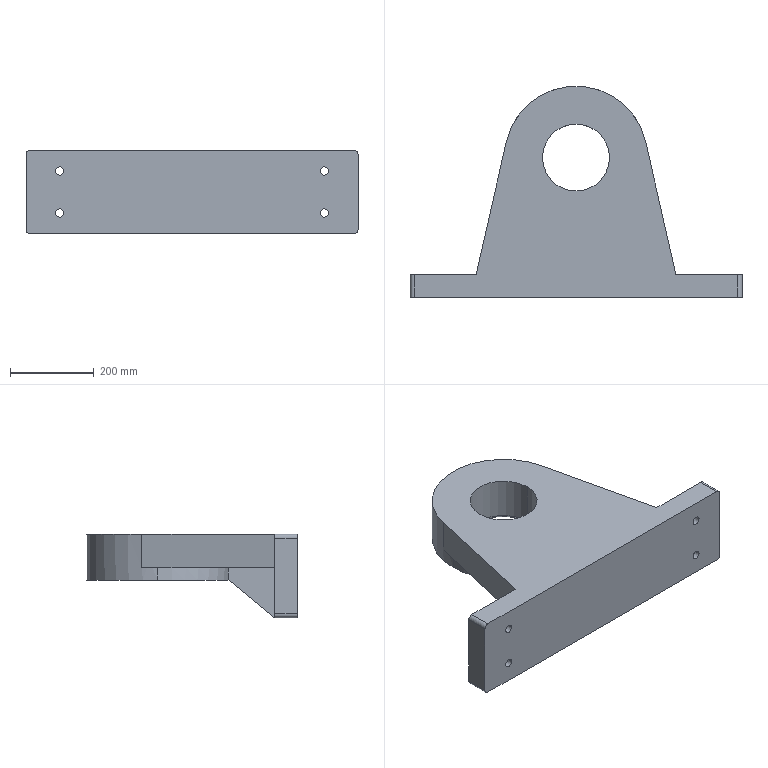Component | SolidWorks | SupportBase-1 | 1 solid | 34 faces | box 792.3 x 503.84 x 200 mm | volume 22321151 mm3 | cylinder 17 | plane 15 | cone 2 | commonest cylinder face diameters 20 x12 340.971 x3 160 x2 | material 45
STEP:
#1=CARTESIAN_POINT('',(57.666,-2.087,-8.071));
#2=VERTEX_POINT('',#1);
#3=CARTESIAN_POINT('',(56.878,-2.087,-8.071));
#4=VERTEX_POINT('',#3);
#5=CARTESIAN_POINT('',(57.272,-2.087,-8.071));
#6=DIRECTION('',(-0.,1.,0.));
#7=DIRECTION('',(-1.,0.,0.));
#8=AXIS2_PLACEMENT_3D('',#5,#6,#7);
#9=CIRCLE('',#8,0.3937);
#10=EDGE_CURVE('',#2,#4,#9,.T.);
#11=ORIENTED_EDGE('',*,*,#10,.F.);
#12=CARTESIAN_POINT('',(57.666,0.04869,-8.071));
#13=VERTEX_POINT('',#12);
#14=CARTESIAN_POINT('',(57.666,-5.424,-8.071));
#15=DIRECTION('',(-0.,1.,0.));
#16=VECTOR('',#15,39.37);
#17=LINE('',#14,#16);
#18=EDGE_CURVE('',#2,#13,#17,.T.);
#19=ORIENTED_EDGE('',*,*,#18,.T.);
#20=CARTESIAN_POINT('',(56.878,0.04869,-8.071));
#21=VERTEX_POINT('',#20);
#22=CARTESIAN_POINT('',(57.272,0.04869,-8.071));
#23=DIRECTION('',(-0.,1.,0.));
#24=DIRECTION('',(-1.,-0.,0.));
#25=AXIS2_PLACEMENT_3D('',#22,#23,#24);
#26=CIRCLE('',#25,0.3937);
#27=EDGE_CURVE('',#13,#21,#26,.T.);
#28=ORIENTED_EDGE('',*,*,#27,.T.);
#29=CARTESIAN_POINT('',(56.878,-5.424,-8.071));
#30=DIRECTION('',(-0.,1.,0.));
#31=VECTOR('',#30,39.37);
#32=LINE('',#29,#31);
#33=EDGE_CURVE('',#4,#21,#32,.T.);
#34=ORIENTED_EDGE('',*,*,#33,.F.);
#35=EDGE_LOOP('',(#11,#19,#28,#34));
#36=FACE_OUTER_BOUND('',#35,.T.);
#37=CARTESIAN_POINT('',(57.272,-5.424,-8.071));
#38=DIRECTION('',(-0.,1.,0.));
#39=DIRECTION('',(-1.,0.,0.));
#40=AXIS2_PLACEMENT_3D('',#37,#38,#39);
#41=CYLINDRICAL_SURFACE('',#40,0.3937);
#42=ADVANCED_FACE('',(#36),#41,.F.);
#43=CARTESIAN_POINT('',(57.666,-2.087,-12.008));
#44=VERTEX_POINT('',#43);
#45=CARTESIAN_POINT('',(56.878,-2.087,-12.008));
#46=VERTEX_POINT('',#45);
#47=CARTESIAN_POINT('',(57.272,-2.087,-12.008));
#48=DIRECTION('',(-0.,1.,0.));
#49=DIRECTION('',(-1.,0.,0.));
#50=AXIS2_PLACEMENT_3D('',#47,#48,#49);
#51=CIRCLE('',#50,0.3937);
#52=EDGE_CURVE('',#44,#46,#51,.T.);
#53=ORIENTED_EDGE('',*,*,#52,.F.);
#54=CARTESIAN_POINT('',(57.666,0.04869,-12.008));
#55=VERTEX_POINT('',#54);
#56=CARTESIAN_POINT('',(57.666,-5.424,-12.008));
#57=DIRECTION('',(-0.,1.,0.));
#58=VECTOR('',#57,39.37);
#59=LINE('',#56,#58);
#60=EDGE_CURVE('',#44,#55,#59,.T.);
#61=ORIENTED_EDGE('',*,*,#60,.T.);
#62=CARTESIAN_POINT('',(56.878,0.04869,-12.008));
#63=VERTEX_POINT('',#62);
#64=CARTESIAN_POINT('',(57.272,0.04869,-12.008));
#65=DIRECTION('',(-0.,1.,0.));
#66=DIRECTION('',(1.,0.,0.));
#67=AXIS2_PLACEMENT_3D('',#64,#65,#66);
#68=CIRCLE('',#67,0.3937);
#69=EDGE_CURVE('',#55,#63,#68,.T.);
#70=ORIENTED_EDGE('',*,*,#69,.T.);
#71=CARTESIAN_POINT('',(56.878,-5.424,-12.008));
#72=DIRECTION('',(-0.,1.,0.));
#73=VECTOR('',#72,39.37);
#74=LINE('',#71,#73);
#75=EDGE_CURVE('',#46,#63,#74,.T.);
#76=ORIENTED_EDGE('',*,*,#75,.F.);
#77=EDGE_LOOP('',(#53,#61,#70,#76));
#78=FACE_OUTER_BOUND('',#77,.T.);
#79=CARTESIAN_POINT('',(57.272,-5.424,-12.008));
#80=DIRECTION('',(-0.,1.,0.));
#81=DIRECTION('',(-1.,0.,0.));
#82=AXIS2_PLACEMENT_3D('',#79,#80,#81);
#83=CYLINDRICAL_SURFACE('',#82,0.3937);
#84=ADVANCED_FACE('',(#78),#83,.F.);
#85=CARTESIAN_POINT('',(32.772,-2.087,-8.071));
#86=VERTEX_POINT('',#85);
#87=CARTESIAN_POINT('',(31.985,-2.087,-8.071));
#88=VERTEX_POINT('',#87);
#89=CARTESIAN_POINT('',(32.378,-2.087,-8.071));
#90=DIRECTION('',(-0.,1.,0.));
#91=DIRECTION('',(-1.,0.,0.));
#92=AXIS2_PLACEMENT_3D('',#89,#90,#91);
#93=CIRCLE('',#92,0.3937);
#94=EDGE_CURVE('',#86,#88,#93,.T.);
#95=ORIENTED_EDGE('',*,*,#94,.F.);
#96=CARTESIAN_POINT('',(32.772,0.04869,-8.071));
#97=VERTEX_POINT('',#96);
#98=CARTESIAN_POINT('',(32.772,-5.424,-8.071));
#99=DIRECTION('',(-0.,1.,0.));
#100=VECTOR('',#99,39.37);
#101=LINE('',#98,#100);
#102=EDGE_CURVE('',#86,#97,#101,.T.);
#103=ORIENTED_EDGE('',*,*,#102,.T.);
#104=CARTESIAN_POINT('',(31.985,0.04869,-8.071));
#105=VERTEX_POINT('',#104);
#106=CARTESIAN_POINT('',(32.378,0.04869,-8.071));
#107=DIRECTION('',(-0.,1.,0.));
#108=DIRECTION('',(1.,0.,0.));
#109=AXIS2_PLACEMENT_3D('',#106,#107,#108);
#110=CIRCLE('',#109,0.3937);
#111=EDGE_CURVE('',#97,#105,#110,.T.);
#112=ORIENTED_EDGE('',*,*,#111,.T.);
#113=CARTESIAN_POINT('',(31.985,-5.424,-8.071));
#114=DIRECTION('',(-0.,1.,0.));
#115=VECTOR('',#114,39.37);
#116=LINE('',#113,#115);
#117=EDGE_CURVE('',#88,#105,#116,.T.);
#118=ORIENTED_EDGE('',*,*,#117,.F.);
#119=EDGE_LOOP('',(#95,#103,#112,#118));
#120=FACE_OUTER_BOUND('',#119,.T.);
#121=CARTESIAN_POINT('',(32.378,-5.424,-8.071));
#122=DIRECTION('',(-0.,1.,0.));
#123=DIRECTION('',(-1.,0.,0.));
#124=AXIS2_PLACEMENT_3D('',#121,#122,#123);
#125=CYLINDRICAL_SURFACE('',#124,0.3937);
#126=ADVANCED_FACE('',(#120),#125,.F.);
#127=CARTESIAN_POINT('',(32.772,-2.087,-12.008));
#128=VERTEX_POINT('',#127);
#129=CARTESIAN_POINT('',(31.985,-2.087,-12.008));
#130=VERTEX_POINT('',#129);
#131=CARTESIAN_POINT('',(32.378,-2.087,-12.008));
#132=DIRECTION('',(-0.,1.,0.));
#133=DIRECTION('',(-1.,0.,0.));
#134=AXIS2_PLACEMENT_3D('',#131,#132,#133);
#135=CIRCLE('',#134,0.3937);
#136=EDGE_CURVE('',#128,#130,#135,.T.);
#137=ORIENTED_EDGE('',*,*,#136,.F.);
#138=CARTESIAN_POINT('',(32.772,0.04869,-12.008));
#139=VERTEX_POINT('',#138);
#140=CARTESIAN_POINT('',(32.772,-5.424,-12.008));
#141=DIRECTION('',(-0.,1.,0.));
#142=VECTOR('',#141,39.37);
#143=LINE('',#140,#142);
#144=EDGE_CURVE('',#128,#139,#143,.T.);
#145=ORIENTED_EDGE('',*,*,#144,.T.);
#146=CARTESIAN_POINT('',(31.985,0.04869,-12.008));
#147=VERTEX_POINT('',#146);
#148=CARTESIAN_POINT('',(32.378,0.04869,-12.008));
#149=DIRECTION('',(-0.,1.,0.));
#150=DIRECTION('',(-1.,-0.,0.));
#151=AXIS2_PLACEMENT_3D('',#148,#149,#150);
#152=CIRCLE('',#151,0.3937);
#153=EDGE_CURVE('',#139,#147,#152,.T.);
#154=ORIENTED_EDGE('',*,*,#153,.T.);
#155=CARTESIAN_POINT('',(31.985,-5.424,-12.008));
#156=DIRECTION('',(-0.,1.,0.));
#157=VECTOR('',#156,39.37);
#158=LINE('',#155,#157);
#159=EDGE_CURVE('',#130,#147,#158,.T.);
#160=ORIENTED_EDGE('',*,*,#159,.F.);
#161=EDGE_LOOP('',(#137,#145,#154,#160));
#162=FACE_OUTER_BOUND('',#161,.T.);
#163=CARTESIAN_POINT('',(32.378,-5.424,-12.008));
#164=DIRECTION('',(-0.,1.,0.));
#165=DIRECTION('',(-1.,0.,0.));
#166=AXIS2_PLACEMENT_3D('',#163,#164,#165);
#167=CYLINDRICAL_SURFACE('',#166,0.3937);
#168=ADVANCED_FACE('',(#162),#167,.F.);
#169=CARTESIAN_POINT('',(47.975,11.038,-10.039));
#170=VERTEX_POINT('',#169);
#171=CARTESIAN_POINT('',(41.676,11.038,-10.039));
#172=VERTEX_POINT('',#171);
#173=CARTESIAN_POINT('',(44.825,11.038,-10.039));
#174=DIRECTION('',(0.,0.,-1.));
#175=DIRECTION('',(-1.,0.,0.));
#176=AXIS2_PLACEMENT_3D('',#173,#174,#175);
#177=CIRCLE('',#176,3.15);
#178=EDGE_CURVE('',#170,#172,#177,.T.);
#179=ORIENTED_EDGE('',*,*,#178,.F.);
#180=CARTESIAN_POINT('',(48.369,11.038,-10.433));
#181=VERTEX_POINT('',#180);
#182=CARTESIAN_POINT('',(47.975,11.038,-10.039));
#183=DIRECTION('',(0.7071,0.,-0.7071));
#184=VECTOR('',#183,39.37);
#185=LINE('',#182,#184);
#186=EDGE_CURVE('',#170,#181,#185,.T.);
#187=ORIENTED_EDGE('',*,*,#186,.T.);
#188=CARTESIAN_POINT('',(41.282,11.038,-10.433));
#189=VERTEX_POINT('',#188);
#190=CARTESIAN_POINT('',(44.825,11.038,-10.433));
#191=DIRECTION('',(0.,0.,1.));
#192=DIRECTION('',(-1.,0.,0.));
#193=AXIS2_PLACEMENT_3D('',#190,#191,#192);
#194=CIRCLE('',#193,3.543);
#195=EDGE_CURVE('',#189,#181,#194,.T.);
#196=ORIENTED_EDGE('',*,*,#195,.F.);
#197=CARTESIAN_POINT('',(41.676,11.038,-10.039));
#198=DIRECTION('',(-0.7071,0.,-0.7071));
#199=VECTOR('',#198,39.37);
#200=LINE('',#197,#199);
#201=EDGE_CURVE('',#172,#189,#200,.T.);
#202=ORIENTED_EDGE('',*,*,#201,.F.);
#203=EDGE_LOOP('',(#179,#187,#196,#202));
#204=FACE_OUTER_BOUND('',#203,.T.);
#205=CARTESIAN_POINT('',(44.825,11.038,-10.039));
#206=DIRECTION('',(0.,0.,-1.));
#207=DIRECTION('',(-1.,0.,0.));
#208=AXIS2_PLACEMENT_3D('',#205,#206,#207);
#209=CONICAL_SURFACE('',#208,3.15,0.7854);
#210=ADVANCED_FACE('',(#204),#209,.F.);
#211=CARTESIAN_POINT('',(41.676,11.038,-6.102));
#212=VERTEX_POINT('',#211);
#213=CARTESIAN_POINT('',(47.975,11.038,-6.102));
#214=VERTEX_POINT('',#213);
#215=CARTESIAN_POINT('',(44.825,11.038,-6.102));
#216=DIRECTION('',(0.,0.,1.));
#217=DIRECTION('',(1.,0.,0.));
#218=AXIS2_PLACEMENT_3D('',#215,#216,#217);
#219=CIRCLE('',#218,3.15);
#220=EDGE_CURVE('',#212,#214,#219,.T.);
#221=ORIENTED_EDGE('',*,*,#220,.T.);
#222=CARTESIAN_POINT('',(47.975,11.038,-6.102));
#223=DIRECTION('',(0.,0.,-1.));
#224=VECTOR('',#223,39.37);
#225=LINE('',#222,#224);
#226=EDGE_CURVE('',#214,#170,#225,.T.);
#227=ORIENTED_EDGE('',*,*,#226,.T.);
#228=ORIENTED_EDGE('',*,*,#178,.T.);
#229=CARTESIAN_POINT('',(41.676,11.038,-6.102));
#230=DIRECTION('',(0.,0.,-1.));
#231=VECTOR('',#230,39.37);
#232=LINE('',#229,#231);
#233=EDGE_CURVE('',#212,#172,#232,.T.);
#234=ORIENTED_EDGE('',*,*,#233,.F.);
#235=EDGE_LOOP('',(#221,#227,#228,#234));
#236=FACE_OUTER_BOUND('',#235,.T.);
#237=CARTESIAN_POINT('',(44.825,11.038,-6.102));
#238=DIRECTION('',(0.,0.,-1.));
#239=DIRECTION('',(-1.,0.,0.));
#240=AXIS2_PLACEMENT_3D('',#237,#238,#239);
#241=CYLINDRICAL_SURFACE('',#240,3.15);
#242=ADVANCED_FACE('',(#236),#241,.F.);
#243=CARTESIAN_POINT('',(51.37,12.528,-9.252));
#244=VERTEX_POINT('',#243);
#245=CARTESIAN_POINT('',(51.537,11.038,-9.252));
#246=VERTEX_POINT('',#245);
#247=CARTESIAN_POINT('',(44.825,11.038,-9.252));
#248=DIRECTION('',(0.,0.,-1.));
#249=DIRECTION('',(1.,0.,0.));
#250=AXIS2_PLACEMENT_3D('',#247,#248,#249);
#251=CIRCLE('',#250,6.712);
#252=EDGE_CURVE('',#244,#246,#251,.T.);
#253=ORIENTED_EDGE('',*,*,#252,.T.);
#254=CARTESIAN_POINT('',(51.537,11.038,-10.433));
#255=VERTEX_POINT('',#254);
#256=CARTESIAN_POINT('',(51.537,11.038,-6.102));
#257=DIRECTION('',(0.,0.,-1.));
#258=VECTOR('',#257,39.37);
#259=LINE('',#256,#258);
#260=EDGE_CURVE('',#246,#255,#259,.T.);
#261=ORIENTED_EDGE('',*,*,#260,.T.);
#262=CARTESIAN_POINT('',(38.113,11.038,-10.433));
#263=VERTEX_POINT('',#262);
#264=CARTESIAN_POINT('',(44.825,11.038,-10.433));
#265=DIRECTION('',(0.,0.,-1.));
#266=DIRECTION('',(-1.,0.,0.));
#267=AXIS2_PLACEMENT_3D('',#264,#265,#266);
#268=CIRCLE('',#267,6.712);
#269=EDGE_CURVE('',#263,#255,#268,.T.);
#270=ORIENTED_EDGE('',*,*,#269,.F.);
#271=CARTESIAN_POINT('',(38.113,11.038,-9.252));
#272=VERTEX_POINT('',#271);
#273=CARTESIAN_POINT('',(38.113,11.038,-6.102));
#274=DIRECTION('',(0.,0.,-1.));
#275=VECTOR('',#274,39.37);
#276=LINE('',#273,#275);
#277=EDGE_CURVE('',#272,#263,#276,.T.);
#278=ORIENTED_EDGE('',*,*,#277,.F.);
#279=CARTESIAN_POINT('',(38.281,12.528,-9.252));
#280=VERTEX_POINT('',#279);
#281=CARTESIAN_POINT('',(44.825,11.038,-9.252));
#282=DIRECTION('',(0.,0.,-1.));
#283=DIRECTION('',(1.,0.,0.));
#284=AXIS2_PLACEMENT_3D('',#281,#282,#283);
#285=CIRCLE('',#284,6.712);
#286=EDGE_CURVE('',#272,#280,#285,.T.);
#287=ORIENTED_EDGE('',*,*,#286,.T.);
#288=CARTESIAN_POINT('',(38.281,12.528,-6.102));
#289=VERTEX_POINT('',#288);
#290=CARTESIAN_POINT('',(38.281,12.528,-6.102));
#291=DIRECTION('',(0.,0.,-1.));
#292=VECTOR('',#291,39.37);
#293=LINE('',#290,#292);
#294=EDGE_CURVE('',#289,#280,#293,.T.);
#295=ORIENTED_EDGE('',*,*,#294,.F.);
#296=CARTESIAN_POINT('',(51.37,12.528,-6.102));
#297=VERTEX_POINT('',#296);
#298=CARTESIAN_POINT('',(44.825,11.038,-6.102));
#299=DIRECTION('',(0.,0.,1.));
#300=DIRECTION('',(1.,0.,0.));
#301=AXIS2_PLACEMENT_3D('',#298,#299,#300);
#302=CIRCLE('',#301,6.712);
#303=EDGE_CURVE('',#297,#289,#302,.T.);
#304=ORIENTED_EDGE('',*,*,#303,.F.);
#305=CARTESIAN_POINT('',(51.37,12.528,-6.102));
#306=DIRECTION('',(0.,0.,-1.));
#307=VECTOR('',#306,39.37);
#308=LINE('',#305,#307);
#309=EDGE_CURVE('',#297,#244,#308,.T.);
#310=ORIENTED_EDGE('',*,*,#309,.T.);
#311=EDGE_LOOP('',(#253,#261,#270,#278,#287,#295,#304,#310));
#312=FACE_OUTER_BOUND('',#311,.T.);
#313=CARTESIAN_POINT('',(44.825,11.038,-6.102));
#314=DIRECTION('',(0.,0.,-1.));
#315=DIRECTION('',(-1.,0.,0.));
#316=AXIS2_PLACEMENT_3D('',#313,#314,#315);
#317=CYLINDRICAL_SURFACE('',#316,6.712);
#318=ADVANCED_FACE('',(#312),#317,.T.);
#319=CARTESIAN_POINT('',(43.841,4.398,-9.252));
#320=VERTEX_POINT('',#319);
#321=CARTESIAN_POINT('',(44.825,11.038,-9.252));
#322=DIRECTION('',(0.,0.,-1.));
#323=DIRECTION('',(1.,0.,0.));
#324=AXIS2_PLACEMENT_3D('',#321,#322,#323);
#325=CIRCLE('',#324,6.712);
#326=EDGE_CURVE('',#320,#272,#325,.T.);
#327=ORIENTED_EDGE('',*,*,#326,.T.);
#328=ORIENTED_EDGE('',*,*,#277,.T.);
#329=CARTESIAN_POINT('',(44.825,4.326,-10.433));
#330=VERTEX_POINT('',#329);
#331=CARTESIAN_POINT('',(44.825,11.038,-10.433));
#332=DIRECTION('',(0.,0.,-1.));
#333=DIRECTION('',(-1.,0.,0.));
#334=AXIS2_PLACEMENT_3D('',#331,#332,#333);
#335=CIRCLE('',#334,6.712);
#336=EDGE_CURVE('',#330,#263,#335,.T.);
#337=ORIENTED_EDGE('',*,*,#336,.F.);
#338=CARTESIAN_POINT('',(43.841,4.398,-10.373));
#339=VERTEX_POINT('',#338);
#340=CARTESIAN_POINT('',(44.825,4.326,-10.433));
#341=CARTESIAN_POINT('',(44.496,4.326,-10.433));
#342=CARTESIAN_POINT('',(44.167,4.35,-10.413));
#343=CARTESIAN_POINT('',(43.841,4.398,-10.373));
#344=(BOUNDED_CURVE()B_SPLINE_CURVE(3,(#340,#341,#342,#343),.UNSPECIFIED.,.F.,.T.)B_SPLINE_CURVE_WITH_KNOTS((4,4),(0.,0.1472),.UNSPECIFIED.)CURVE()GEOMETRIC_REPRESENTATION_ITEM()RATIONAL_B_SPLINE_CURVE((1.,0.9982,0.9982,1.))REPRESENTATION_ITEM(''));
#345=EDGE_CURVE('',#330,#339,#344,.T.);
#346=ORIENTED_EDGE('',*,*,#345,.T.);
#347=CARTESIAN_POINT('',(43.841,4.398,-6.102));
#348=DIRECTION('',(0.,0.,1.));
#349=VECTOR('',#348,39.37);
#350=LINE('',#347,#349);
#351=EDGE_CURVE('',#339,#320,#350,.T.);
#352=ORIENTED_EDGE('',*,*,#351,.T.);
#353=EDGE_LOOP('',(#327,#328,#337,#346,#352));
#354=FACE_OUTER_BOUND('',#353,.T.);
#355=CARTESIAN_POINT('',(44.825,11.038,-6.102));
#356=DIRECTION('',(0.,0.,-1.));
#357=DIRECTION('',(-1.,0.,0.));
#358=AXIS2_PLACEMENT_3D('',#355,#356,#357);
#359=CYLINDRICAL_SURFACE('',#358,6.712);
#360=ADVANCED_FACE('',(#354),#359,.T.);
#361=CARTESIAN_POINT('',(45.81,4.398,-9.252));
#362=VERTEX_POINT('',#361);
#363=CARTESIAN_POINT('',(45.81,0.04869,-9.252));
#364=VERTEX_POINT('',#363);
#365=CARTESIAN_POINT('',(45.81,0.01034,-9.252));
#366=DIRECTION('',(0.,-1.,0.));
#367=VECTOR('',#366,39.37);
#368=LINE('',#365,#367);
#369=EDGE_CURVE('',#362,#364,#368,.T.);
#370=ORIENTED_EDGE('',*,*,#369,.F.);
#371=CARTESIAN_POINT('',(44.825,11.038,-9.252));
#372=DIRECTION('',(0.,0.,-1.));
#373=DIRECTION('',(1.,0.,0.));
#374=AXIS2_PLACEMENT_3D('',#371,#372,#373);
#375=CIRCLE('',#374,6.712);
#376=EDGE_CURVE('',#246,#362,#375,.T.);
#377=ORIENTED_EDGE('',*,*,#376,.F.);
#378=ORIENTED_EDGE('',*,*,#252,.F.);
#379=CARTESIAN_POINT('',(54.213,0.04869,-9.252));
#380=VERTEX_POINT('',#379);
#381=CARTESIAN_POINT('',(51.816,10.571,-9.252));
#382=DIRECTION('',(-0.2221,0.975,0.));
#383=VECTOR('',#382,39.37);
#384=LINE('',#381,#383);
#385=EDGE_CURVE('',#380,#244,#384,.T.);
#386=ORIENTED_EDGE('',*,*,#385,.F.);
#387=CARTESIAN_POINT('',(5.455,0.04869,-9.252));
#388=DIRECTION('',(-1.,0.,0.));
#389=VECTOR('',#388,39.37);
#390=LINE('',#387,#389);
#391=EDGE_CURVE('',#380,#364,#390,.T.);
#392=ORIENTED_EDGE('',*,*,#391,.T.);
#393=EDGE_LOOP('',(#370,#377,#378,#386,#392));
#394=FACE_OUTER_BOUND('',#393,.T.);
#395=CARTESIAN_POINT('',(5.455,0.01034,-9.252));
#396=DIRECTION('',(0.,0.,1.));
#397=DIRECTION('',(1.,0.,0.));
#398=AXIS2_PLACEMENT_3D('',#395,#396,#397);
#399=PLANE('',#398);
#400=ADVANCED_FACE('',(#394),#399,.F.);
#401=CARTESIAN_POINT('',(57.272,0.04869,-8.071));
#402=DIRECTION('',(-0.,1.,0.));
#403=DIRECTION('',(-1.,-0.,0.));
#404=AXIS2_PLACEMENT_3D('',#401,#402,#403);
#405=CIRCLE('',#404,0.3937);
#406=EDGE_CURVE('',#21,#13,#405,.T.);
#407=ORIENTED_EDGE('',*,*,#406,.F.);
#408=ORIENTED_EDGE('',*,*,#27,.F.);
#409=EDGE_LOOP('',(#407,#408));
#410=FACE_BOUND('',#409,.T.);
#411=CARTESIAN_POINT('',(57.272,0.04869,-12.008));
#412=DIRECTION('',(-0.,1.,0.));
#413=DIRECTION('',(1.,0.,0.));
#414=AXIS2_PLACEMENT_3D('',#411,#412,#413);
#415=CIRCLE('',#414,0.3937);
#416=EDGE_CURVE('',#63,#55,#415,.T.);
#417=ORIENTED_EDGE('',*,*,#416,.F.);
#418=ORIENTED_EDGE('',*,*,#69,.F.);
#419=EDGE_LOOP('',(#417,#418));
#420=FACE_BOUND('',#419,.T.);
#421=CARTESIAN_POINT('',(60.028,0.04869,-6.102));
#422=VERTEX_POINT('',#421);
#423=CARTESIAN_POINT('',(54.213,0.04869,-6.102));
#424=VERTEX_POINT('',#423);
#425=CARTESIAN_POINT('',(5.455,0.04869,-6.102));
#426=DIRECTION('',(-1.,-0.,0.));
#427=VECTOR('',#426,39.37);
#428=LINE('',#425,#427);
#429=EDGE_CURVE('',#422,#424,#428,.T.);
#430=ORIENTED_EDGE('',*,*,#429,.F.);
#431=CARTESIAN_POINT('',(60.422,0.04869,-6.496));
#432=VERTEX_POINT('',#431);
#433=CARTESIAN_POINT('',(60.028,0.04869,-6.496));
#434=DIRECTION('',(-0.,1.,0.));
#435=DIRECTION('',(1.,0.,0.));
#436=AXIS2_PLACEMENT_3D('',#433,#434,#435);
#437=CIRCLE('',#436,0.3937);
#438=EDGE_CURVE('',#422,#432,#437,.T.);
#439=ORIENTED_EDGE('',*,*,#438,.T.);
#440=CARTESIAN_POINT('',(60.422,0.04869,-13.583));
#441=VERTEX_POINT('',#440);
#442=CARTESIAN_POINT('',(60.422,0.04869,-6.102));
#443=DIRECTION('',(0.,0.,-1.));
#444=VECTOR('',#443,39.37);
#445=LINE('',#442,#444);
#446=EDGE_CURVE('',#432,#441,#445,.T.);
#447=ORIENTED_EDGE('',*,*,#446,.T.);
#448=CARTESIAN_POINT('',(60.028,0.04869,-13.976));
#449=VERTEX_POINT('',#448);
#450=CARTESIAN_POINT('',(60.028,0.04869,-13.583));
#451=DIRECTION('',(-0.,1.,0.));
#452=DIRECTION('',(1.,0.,0.));
#453=AXIS2_PLACEMENT_3D('',#450,#451,#452);
#454=CIRCLE('',#453,0.3937);
#455=EDGE_CURVE('',#441,#449,#454,.T.);
#456=ORIENTED_EDGE('',*,*,#455,.T.);
#457=CARTESIAN_POINT('',(45.81,0.04869,-13.976));
#458=VERTEX_POINT('',#457);
#459=CARTESIAN_POINT('',(29.229,0.04869,-13.976));
#460=DIRECTION('',(-1.,0.,0.));
#461=VECTOR('',#460,39.37);
#462=LINE('',#459,#461);
#463=EDGE_CURVE('',#449,#458,#462,.T.);
#464=ORIENTED_EDGE('',*,*,#463,.T.);
#465=CARTESIAN_POINT('',(45.81,0.04869,-6.102));
#466=DIRECTION('',(0.,0.,-1.));
#467=VECTOR('',#466,39.37);
#468=LINE('',#465,#467);
#469=EDGE_CURVE('',#364,#458,#468,.T.);
#470=ORIENTED_EDGE('',*,*,#469,.F.);
#471=ORIENTED_EDGE('',*,*,#391,.F.);
#472=CARTESIAN_POINT('',(54.213,0.04869,-6.102));
#473=DIRECTION('',(0.,0.,-1.));
#474=VECTOR('',#473,39.37);
#475=LINE('',#472,#474);
#476=EDGE_CURVE('',#424,#380,#475,.T.);
#477=ORIENTED_EDGE('',*,*,#476,.F.);
#478=EDGE_LOOP('',(#430,#439,#447,#456,#464,#470,#471,#477));
#479=FACE_OUTER_BOUND('',#478,.T.);
#480=CARTESIAN_POINT('',(5.455,0.04869,-6.102));
#481=DIRECTION('',(0.,-1.,0.));
#482=DIRECTION('',(1.,0.,0.));
#483=AXIS2_PLACEMENT_3D('',#480,#481,#482);
#484=PLANE('',#483);
#485=ADVANCED_FACE('',(#410,#420,#479),#484,.F.);
#486=ORIENTED_EDGE('',*,*,#326,.F.);
#487=CARTESIAN_POINT('',(43.841,0.04869,-9.252));
#488=VERTEX_POINT('',#487);
#489=CARTESIAN_POINT('',(43.841,0.01034,-9.252));
#490=DIRECTION('',(0.,-1.,0.));
#491=VECTOR('',#490,39.37);
#492=LINE('',#489,#491);
#493=EDGE_CURVE('',#320,#488,#492,.T.);
#494=ORIENTED_EDGE('',*,*,#493,.T.);
#495=CARTESIAN_POINT('',(35.438,0.04869,-9.252));
#496=VERTEX_POINT('',#495);
#497=CARTESIAN_POINT('',(5.455,0.04869,-9.252));
#498=DIRECTION('',(-1.,0.,0.));
#499=VECTOR('',#498,39.37);
#500=LINE('',#497,#499);
#501=EDGE_CURVE('',#488,#496,#500,.T.);
#502=ORIENTED_EDGE('',*,*,#501,.T.);
#503=CARTESIAN_POINT('',(33.951,-6.481,-9.252));
#504=DIRECTION('',(0.2221,0.975,0.));
#505=VECTOR('',#504,39.37);
#506=LINE('',#503,#505);
#507=EDGE_CURVE('',#496,#280,#506,.T.);
#508=ORIENTED_EDGE('',*,*,#507,.T.);
#509=ORIENTED_EDGE('',*,*,#286,.F.);
#510=EDGE_LOOP('',(#486,#494,#502,#508,#509));
#511=FACE_OUTER_BOUND('',#510,.T.);
#512=CARTESIAN_POINT('',(5.455,0.01034,-9.252));
#513=DIRECTION('',(0.,0.,1.));
#514=DIRECTION('',(1.,0.,0.));
#515=AXIS2_PLACEMENT_3D('',#512,#513,#514);
#516=PLANE('',#515);
#517=ADVANCED_FACE('',(#511),#516,.F.);
#518=ORIENTED_EDGE('',*,*,#260,.F.);
#519=ORIENTED_EDGE('',*,*,#376,.T.);
#520=CARTESIAN_POINT('',(45.81,4.398,-10.373));
#521=VERTEX_POINT('',#520);
#522=CARTESIAN_POINT('',(45.81,4.398,-6.102));
#523=DIRECTION('',(0.,0.,1.));
#524=VECTOR('',#523,39.37);
#525=LINE('',#522,#524);
#526=EDGE_CURVE('',#521,#362,#525,.T.);
#527=ORIENTED_EDGE('',*,*,#526,.F.);
#528=CARTESIAN_POINT('',(45.81,4.398,-10.373));
#529=CARTESIAN_POINT('',(45.484,4.35,-10.413));
#530=CARTESIAN_POINT('',(45.155,4.326,-10.433));
#531=CARTESIAN_POINT('',(44.825,4.326,-10.433));
#532=(BOUNDED_CURVE()B_SPLINE_CURVE(3,(#528,#529,#530,#531),.UNSPECIFIED.,.F.,.T.)B_SPLINE_CURVE_WITH_KNOTS((4,4),(6.136,6.283),.UNSPECIFIED.)CURVE()GEOMETRIC_REPRESENTATION_ITEM()RATIONAL_B_SPLINE_CURVE((1.,0.9982,0.9982,1.))REPRESENTATION_ITEM(''));
#533=EDGE_CURVE('',#521,#330,#532,.T.);
#534=ORIENTED_EDGE('',*,*,#533,.T.);
#535=CARTESIAN_POINT('',(44.825,11.038,-10.433));
#536=DIRECTION('',(0.,0.,-1.));
#537=DIRECTION('',(-1.,0.,0.));
#538=AXIS2_PLACEMENT_3D('',#535,#536,#537);
#539=CIRCLE('',#538,6.712);
#540=EDGE_CURVE('',#255,#330,#539,.T.);
#541=ORIENTED_EDGE('',*,*,#540,.F.);
#542=EDGE_LOOP('',(#518,#519,#527,#534,#541));
#543=FACE_OUTER_BOUND('',#542,.T.);
#544=CARTESIAN_POINT('',(44.825,11.038,-6.102));
#545=DIRECTION('',(0.,0.,-1.));
#546=DIRECTION('',(-1.,0.,0.));
#547=AXIS2_PLACEMENT_3D('',#544,#545,#546);
#548=CYLINDRICAL_SURFACE('',#547,6.712);
#549=ADVANCED_FACE('',(#543),#548,.T.);
#550=ORIENTED_EDGE('',*,*,#507,.F.);
#551=CARTESIAN_POINT('',(35.438,0.04869,-6.102));
#552=VERTEX_POINT('',#551);
#553=CARTESIAN_POINT('',(35.438,0.04869,-6.102));
#554=DIRECTION('',(0.,0.,-1.));
#555=VECTOR('',#554,39.37);
#556=LINE('',#553,#555);
#557=EDGE_CURVE('',#552,#496,#556,.T.);
#558=ORIENTED_EDGE('',*,*,#557,.F.);
#559=CARTESIAN_POINT('',(33.951,-6.481,-6.102));
#560=DIRECTION('',(0.2221,0.975,0.));
#561=VECTOR('',#560,39.37);
#562=LINE('',#559,#561);
#563=EDGE_CURVE('',#552,#289,#562,.T.);
#564=ORIENTED_EDGE('',*,*,#563,.T.);
#565=ORIENTED_EDGE('',*,*,#294,.T.);
#566=EDGE_LOOP('',(#550,#558,#564,#565));
#567=FACE_OUTER_BOUND('',#566,.T.);
#568=CARTESIAN_POINT('',(33.951,-6.481,-6.102));
#569=DIRECTION('',(-0.975,0.2221,0.));
#570=DIRECTION('',(-0.2221,-0.975,0.));
#571=AXIS2_PLACEMENT_3D('',#568,#569,#570);
#572=PLANE('',#571);
#573=ADVANCED_FACE('',(#567),#572,.T.);
#574=CARTESIAN_POINT('',(29.229,-2.087,-6.496));
#575=VERTEX_POINT('',#574);
#576=CARTESIAN_POINT('',(29.229,-2.087,-13.583));
#577=VERTEX_POINT('',#576);
#578=CARTESIAN_POINT('',(29.229,-2.087,-6.102));
#579=DIRECTION('',(0.,0.,-1.));
#580=VECTOR('',#579,39.37);
#581=LINE('',#578,#580);
#582=EDGE_CURVE('',#575,#577,#581,.T.);
#583=ORIENTED_EDGE('',*,*,#582,.F.);
#584=CARTESIAN_POINT('',(29.229,0.04869,-6.496));
#585=VERTEX_POINT('',#584);
#586=CARTESIAN_POINT('',(29.229,0.01034,-6.496));
#587=DIRECTION('',(0.,1.,0.));
#588=VECTOR('',#587,39.37);
#589=LINE('',#586,#588);
#590=EDGE_CURVE('',#575,#585,#589,.T.);
#591=ORIENTED_EDGE('',*,*,#590,.T.);
#592=CARTESIAN_POINT('',(29.229,0.04869,-13.583));
#593=VERTEX_POINT('',#592);
#594=CARTESIAN_POINT('',(29.229,0.04869,-6.102));
#595=DIRECTION('',(0.,0.,-1.));
#596=VECTOR('',#595,39.37);
#597=LINE('',#594,#596);
#598=EDGE_CURVE('',#585,#593,#597,.T.);
#599=ORIENTED_EDGE('',*,*,#598,.T.);
#600=CARTESIAN_POINT('',(29.229,-2.087,-13.583));
#601=DIRECTION('',(0.,-1.,0.));
#602=VECTOR('',#601,39.37);
#603=LINE('',#600,#602);
#604=EDGE_CURVE('',#593,#577,#603,.T.);
#605=ORIENTED_EDGE('',*,*,#604,.T.);
#606=EDGE_LOOP('',(#583,#591,#599,#605));
#607=FACE_OUTER_BOUND('',#606,.T.);
#608=CARTESIAN_POINT('',(29.229,0.01034,-6.102));
#609=DIRECTION('',(-1.,0.,0.));
#610=DIRECTION('',(0.,0.,1.));
#611=AXIS2_PLACEMENT_3D('',#608,#609,#610);
#612=PLANE('',#611);
#613=ADVANCED_FACE('',(#607),#612,.T.);
#614=CARTESIAN_POINT('',(32.378,-2.087,-8.071));
#615=DIRECTION('',(-0.,1.,0.));
#616=DIRECTION('',(-1.,0.,0.));
#617=AXIS2_PLACEMENT_3D('',#614,#615,#616);
#618=CIRCLE('',#617,0.3937);
#619=EDGE_CURVE('',#88,#86,#618,.T.);
#620=ORIENTED_EDGE('',*,*,#619,.T.);
#621=ORIENTED_EDGE('',*,*,#94,.T.);
#622=EDGE_LOOP('',(#620,#621));
#623=FACE_BOUND('',#622,.T.);
#624=CARTESIAN_POINT('',(57.272,-2.087,-8.071));
#625=DIRECTION('',(-0.,1.,0.));
#626=DIRECTION('',(-1.,0.,0.));
#627=AXIS2_PLACEMENT_3D('',#624,#625,#626);
#628=CIRCLE('',#627,0.3937);
#629=EDGE_CURVE('',#4,#2,#628,.T.);
#630=ORIENTED_EDGE('',*,*,#629,.T.);
#631=ORIENTED_EDGE('',*,*,#10,.T.);
#632=EDGE_LOOP('',(#630,#631));
#633=FACE_BOUND('',#632,.T.);
#634=CARTESIAN_POINT('',(57.272,-2.087,-12.008));
#635=DIRECTION('',(-0.,1.,0.));
#636=DIRECTION('',(-1.,0.,0.));
#637=AXIS2_PLACEMENT_3D('',#634,#635,#636);
#638=CIRCLE('',#637,0.3937);
#639=EDGE_CURVE('',#46,#44,#638,.T.);
#640=ORIENTED_EDGE('',*,*,#639,.T.);
#641=ORIENTED_EDGE('',*,*,#52,.T.);
#642=EDGE_LOOP('',(#640,#641));
#643=FACE_BOUND('',#642,.T.);
#644=CARTESIAN_POINT('',(32.378,-2.087,-12.008));
#645=DIRECTION('',(-0.,1.,0.));
#646=DIRECTION('',(-1.,0.,0.));
#647=AXIS2_PLACEMENT_3D('',#644,#645,#646);
#648=CIRCLE('',#647,0.3937);
#649=EDGE_CURVE('',#130,#128,#648,.T.);
#650=ORIENTED_EDGE('',*,*,#649,.T.);
#651=ORIENTED_EDGE('',*,*,#136,.T.);
#652=EDGE_LOOP('',(#650,#651));
#653=FACE_BOUND('',#652,.T.);
#654=CARTESIAN_POINT('',(60.422,-2.087,-6.496));
#655=VERTEX_POINT('',#654);
#656=CARTESIAN_POINT('',(60.422,-2.087,-13.583));
#657=VERTEX_POINT('',#656);
#658=CARTESIAN_POINT('',(60.422,-2.087,-6.102));
#659=DIRECTION('',(0.,0.,-1.));
#660=VECTOR('',#659,39.37);
#661=LINE('',#658,#660);
#662=EDGE_CURVE('',#655,#657,#661,.T.);
#663=ORIENTED_EDGE('',*,*,#662,.F.);
#664=CARTESIAN_POINT('',(60.028,-2.087,-6.102));
#665=VERTEX_POINT('',#664);
#666=CARTESIAN_POINT('',(60.028,-2.087,-6.496));
#667=DIRECTION('',(0.,-1.,0.));
#668=DIRECTION('',(-1.,0.,0.));
#669=AXIS2_PLACEMENT_3D('',#666,#667,#668);
#670=CIRCLE('',#669,0.3937);
#671=EDGE_CURVE('',#655,#665,#670,.T.);
#672=ORIENTED_EDGE('',*,*,#671,.T.);
#673=CARTESIAN_POINT('',(29.623,-2.087,-6.102));
#674=VERTEX_POINT('',#673);
#675=CARTESIAN_POINT('',(5.455,-2.087,-6.102));
#676=DIRECTION('',(1.,0.,0.));
#677=VECTOR('',#676,39.37);
#678=LINE('',#675,#677);
#679=EDGE_CURVE('',#674,#665,#678,.T.);
#680=ORIENTED_EDGE('',*,*,#679,.F.);
#681=CARTESIAN_POINT('',(29.623,-2.087,-6.496));
#682=DIRECTION('',(0.,-1.,0.));
#683=DIRECTION('',(-1.,0.,0.));
#684=AXIS2_PLACEMENT_3D('',#681,#682,#683);
#685=CIRCLE('',#684,0.3937);
#686=EDGE_CURVE('',#674,#575,#685,.T.);
#687=ORIENTED_EDGE('',*,*,#686,.T.);
#688=ORIENTED_EDGE('',*,*,#582,.T.);
#689=CARTESIAN_POINT('',(29.623,-2.087,-13.976));
#690=VERTEX_POINT('',#689);
#691=CARTESIAN_POINT('',(29.623,-2.087,-13.583));
#692=DIRECTION('',(0.,-1.,0.));
#693=DIRECTION('',(-1.,0.,0.));
#694=AXIS2_PLACEMENT_3D('',#691,#692,#693);
#695=CIRCLE('',#694,0.3937);
#696=EDGE_CURVE('',#577,#690,#695,.T.);
#697=ORIENTED_EDGE('',*,*,#696,.T.);
#698=CARTESIAN_POINT('',(60.028,-2.087,-13.976));
#699=VERTEX_POINT('',#698);
#700=CARTESIAN_POINT('',(29.229,-2.087,-13.976));
#701=DIRECTION('',(1.,0.,0.));
#702=VECTOR('',#701,39.37);
#703=LINE('',#700,#702);
#704=EDGE_CURVE('',#690,#699,#703,.T.);
#705=ORIENTED_EDGE('',*,*,#704,.T.);
#706=CARTESIAN_POINT('',(60.028,-2.087,-13.583));
#707=DIRECTION('',(0.,-1.,0.));
#708=DIRECTION('',(-1.,0.,0.));
#709=AXIS2_PLACEMENT_3D('',#706,#707,#708);
#710=CIRCLE('',#709,0.3937);
#711=EDGE_CURVE('',#699,#657,#710,.T.);
#712=ORIENTED_EDGE('',*,*,#711,.T.);
#713=EDGE_LOOP('',(#663,#672,#680,#687,#688,#697,#705,#712));
#714=FACE_OUTER_BOUND('',#713,.T.);
#715=CARTESIAN_POINT('',(5.455,-2.087,-6.102));
#716=DIRECTION('',(-0.,1.,0.));
#717=DIRECTION('',(-1.,-0.,0.));
#718=AXIS2_PLACEMENT_3D('',#715,#716,#717);
#719=PLANE('',#718);
#720=ADVANCED_FACE('',(#623,#633,#643,#653,#714),#719,.F.);
#721=ORIENTED_EDGE('',*,*,#446,.F.);
#722=CARTESIAN_POINT('',(60.422,-2.087,-6.496));
#723=DIRECTION('',(0.,-1.,0.));
#724=VECTOR('',#723,39.37);
#725=LINE('',#722,#724);
#726=EDGE_CURVE('',#432,#655,#725,.T.);
#727=ORIENTED_EDGE('',*,*,#726,.T.);
#728=ORIENTED_EDGE('',*,*,#662,.T.);
#729=CARTESIAN_POINT('',(60.422,0.01034,-13.583));
#730=DIRECTION('',(0.,1.,0.));
#731=VECTOR('',#730,39.37);
#732=LINE('',#729,#731);
#733=EDGE_CURVE('',#657,#441,#732,.T.);
#734=ORIENTED_EDGE('',*,*,#733,.T.);
#735=EDGE_LOOP('',(#721,#727,#728,#734));
#736=FACE_OUTER_BOUND('',#735,.T.);
#737=CARTESIAN_POINT('',(60.422,0.01034,-6.102));
#738=DIRECTION('',(-1.,0.,0.));
#739=DIRECTION('',(0.,0.,1.));
#740=AXIS2_PLACEMENT_3D('',#737,#738,#739);
#741=PLANE('',#740);
#742=ADVANCED_FACE('',(#736),#741,.F.);
#743=CARTESIAN_POINT('',(32.378,0.04869,-8.071));
#744=DIRECTION('',(-0.,1.,0.));
#745=DIRECTION('',(1.,0.,0.));
#746=AXIS2_PLACEMENT_3D('',#743,#744,#745);
#747=CIRCLE('',#746,0.3937);
#748=EDGE_CURVE('',#105,#97,#747,.T.);
#749=ORIENTED_EDGE('',*,*,#748,.F.);
#750=ORIENTED_EDGE('',*,*,#111,.F.);
#751=EDGE_LOOP('',(#749,#750));
#752=FACE_BOUND('',#751,.T.);
#753=CARTESIAN_POINT('',(32.378,0.04869,-12.008));
#754=DIRECTION('',(-0.,1.,0.));
#755=DIRECTION('',(-1.,-0.,0.));
#756=AXIS2_PLACEMENT_3D('',#753,#754,#755);
#757=CIRCLE('',#756,0.3937);
#758=EDGE_CURVE('',#147,#139,#757,.T.);
#759=ORIENTED_EDGE('',*,*,#758,.F.);
#760=ORIENTED_EDGE('',*,*,#153,.F.);
#761=EDGE_LOOP('',(#759,#760));
#762=FACE_BOUND('',#761,.T.);
#763=ORIENTED_EDGE('',*,*,#598,.F.);
#764=CARTESIAN_POINT('',(29.623,0.04869,-6.102));
#765=VERTEX_POINT('',#764);
#766=CARTESIAN_POINT('',(29.623,0.04869,-6.496));
#767=DIRECTION('',(-0.,1.,0.));
#768=DIRECTION('',(1.,0.,0.));
#769=AXIS2_PLACEMENT_3D('',#766,#767,#768);
#770=CIRCLE('',#769,0.3937);
#771=EDGE_CURVE('',#585,#765,#770,.T.);
#772=ORIENTED_EDGE('',*,*,#771,.T.);
#773=CARTESIAN_POINT('',(5.455,0.04869,-6.102));
#774=DIRECTION('',(1.,0.,0.));
#775=VECTOR('',#774,39.37);
#776=LINE('',#773,#775);
#777=EDGE_CURVE('',#765,#552,#776,.T.);
#778=ORIENTED_EDGE('',*,*,#777,.T.);
#779=ORIENTED_EDGE('',*,*,#557,.T.);
#780=ORIENTED_EDGE('',*,*,#501,.F.);
#781=CARTESIAN_POINT('',(43.841,0.04869,-13.976));
#782=VERTEX_POINT('',#781);
#783=CARTESIAN_POINT('',(43.841,0.04869,-6.102));
#784=DIRECTION('',(0.,0.,-1.));
#785=VECTOR('',#784,39.37);
#786=LINE('',#783,#785);
#787=EDGE_CURVE('',#488,#782,#786,.T.);
#788=ORIENTED_EDGE('',*,*,#787,.T.);
#789=CARTESIAN_POINT('',(29.623,0.04869,-13.976));
#790=VERTEX_POINT('',#789);
#791=CARTESIAN_POINT('',(29.229,0.04869,-13.976));
#792=DIRECTION('',(-1.,0.,0.));
#793=VECTOR('',#792,39.37);
#794=LINE('',#791,#793);
#795=EDGE_CURVE('',#782,#790,#794,.T.);
#796=ORIENTED_EDGE('',*,*,#795,.T.);
#797=CARTESIAN_POINT('',(29.623,0.04869,-13.583));
#798=DIRECTION('',(-0.,1.,0.));
#799=DIRECTION('',(1.,0.,0.));
#800=AXIS2_PLACEMENT_3D('',#797,#798,#799);
#801=CIRCLE('',#800,0.3937);
#802=EDGE_CURVE('',#790,#593,#801,.T.);
#803=ORIENTED_EDGE('',*,*,#802,.T.);
#804=EDGE_LOOP('',(#763,#772,#778,#779,#780,#788,#796,#803));
#805=FACE_OUTER_BOUND('',#804,.T.);
#806=CARTESIAN_POINT('',(5.455,0.04869,-6.102));
#807=DIRECTION('',(0.,-1.,0.));
#808=DIRECTION('',(1.,0.,0.));
#809=AXIS2_PLACEMENT_3D('',#806,#807,#808);
#810=PLANE('',#809);
#811=ADVANCED_FACE('',(#752,#762,#805),#810,.F.);
#812=ORIENTED_EDGE('',*,*,#226,.F.);
#813=CARTESIAN_POINT('',(44.825,11.038,-6.102));
#814=DIRECTION('',(0.,0.,1.));
#815=DIRECTION('',(1.,0.,0.));
#816=AXIS2_PLACEMENT_3D('',#813,#814,#815);
#817=CIRCLE('',#816,3.15);
#818=EDGE_CURVE('',#214,#212,#817,.T.);
#819=ORIENTED_EDGE('',*,*,#818,.T.);
#820=ORIENTED_EDGE('',*,*,#233,.T.);
#821=CARTESIAN_POINT('',(44.825,11.038,-10.039));
#822=DIRECTION('',(0.,0.,-1.));
#823=DIRECTION('',(-1.,0.,0.));
#824=AXIS2_PLACEMENT_3D('',#821,#822,#823);
#825=CIRCLE('',#824,3.15);
#826=EDGE_CURVE('',#172,#170,#825,.T.);
#827=ORIENTED_EDGE('',*,*,#826,.T.);
#828=EDGE_LOOP('',(#812,#819,#820,#827));
#829=FACE_OUTER_BOUND('',#828,.T.);
#830=CARTESIAN_POINT('',(44.825,11.038,-6.102));
#831=DIRECTION('',(0.,0.,-1.));
#832=DIRECTION('',(-1.,0.,0.));
#833=AXIS2_PLACEMENT_3D('',#830,#831,#832);
#834=CYLINDRICAL_SURFACE('',#833,3.15);
#835=ADVANCED_FACE('',(#829),#834,.F.);
#836=ORIENTED_EDGE('',*,*,#385,.T.);
#837=ORIENTED_EDGE('',*,*,#309,.F.);
#838=CARTESIAN_POINT('',(51.816,10.571,-6.102));
#839=DIRECTION('',(-0.2221,0.975,0.));
#840=VECTOR('',#839,39.37);
#841=LINE('',#838,#840);
#842=EDGE_CURVE('',#424,#297,#841,.T.);
#843=ORIENTED_EDGE('',*,*,#842,.F.);
#844=ORIENTED_EDGE('',*,*,#476,.T.);
#845=EDGE_LOOP('',(#836,#837,#843,#844));
#846=FACE_OUTER_BOUND('',#845,.T.);
#847=CARTESIAN_POINT('',(51.816,10.571,-6.102));
#848=DIRECTION('',(-0.975,-0.2221,0.));
#849=DIRECTION('',(0.2221,-0.975,0.));
#850=AXIS2_PLACEMENT_3D('',#847,#848,#849);
#851=PLANE('',#850);
#852=ADVANCED_FACE('',(#846),#851,.F.);
#853=ORIENTED_EDGE('',*,*,#679,.T.);
#854=CARTESIAN_POINT('',(60.028,0.04869,-6.102));
#855=DIRECTION('',(0.,1.,0.));
#856=VECTOR('',#855,39.37);
#857=LINE('',#854,#856);
#858=EDGE_CURVE('',#665,#422,#857,.T.);
#859=ORIENTED_EDGE('',*,*,#858,.T.);
#860=ORIENTED_EDGE('',*,*,#429,.T.);
#861=ORIENTED_EDGE('',*,*,#842,.T.);
#862=ORIENTED_EDGE('',*,*,#303,.T.);
#863=ORIENTED_EDGE('',*,*,#563,.F.);
#864=ORIENTED_EDGE('',*,*,#777,.F.);
#865=CARTESIAN_POINT('',(29.623,0.01034,-6.102));
#866=DIRECTION('',(0.,-1.,0.));
#867=VECTOR('',#866,39.37);
#868=LINE('',#865,#867);
#869=EDGE_CURVE('',#765,#674,#868,.T.);
#870=ORIENTED_EDGE('',*,*,#869,.T.);
#871=EDGE_LOOP('',(#853,#859,#860,#861,#862,#863,#864,#870));
#872=FACE_OUTER_BOUND('',#871,.T.);
#873=ORIENTED_EDGE('',*,*,#220,.F.);
#874=ORIENTED_EDGE('',*,*,#818,.F.);
#875=EDGE_LOOP('',(#873,#874));
#876=FACE_BOUND('',#875,.T.);
#877=CARTESIAN_POINT('',(5.455,0.01034,-6.102));
#878=DIRECTION('',(0.,0.,1.));
#879=DIRECTION('',(1.,0.,0.));
#880=AXIS2_PLACEMENT_3D('',#877,#878,#879);
#881=PLANE('',#880);
#882=ADVANCED_FACE('',(#872,#876),#881,.T.);
#883=ORIENTED_EDGE('',*,*,#704,.F.);
#884=CARTESIAN_POINT('',(29.623,0.04869,-13.976));
#885=DIRECTION('',(0.,1.,0.));
#886=VECTOR('',#885,39.37);
#887=LINE('',#884,#886);
#888=EDGE_CURVE('',#690,#790,#887,.T.);
#889=ORIENTED_EDGE('',*,*,#888,.T.);
#890=ORIENTED_EDGE('',*,*,#795,.F.);
#891=CARTESIAN_POINT('',(5.455,0.04869,-13.976));
#892=DIRECTION('',(-1.,0.,0.));
#893=VECTOR('',#892,39.37);
#894=LINE('',#891,#893);
#895=EDGE_CURVE('',#458,#782,#894,.T.);
#896=ORIENTED_EDGE('',*,*,#895,.F.);
#897=ORIENTED_EDGE('',*,*,#463,.F.);
#898=CARTESIAN_POINT('',(60.028,0.01034,-13.976));
#899=DIRECTION('',(0.,-1.,0.));
#900=VECTOR('',#899,39.37);
#901=LINE('',#898,#900);
#902=EDGE_CURVE('',#449,#699,#901,.T.);
#903=ORIENTED_EDGE('',*,*,#902,.T.);
#904=EDGE_LOOP('',(#883,#889,#890,#896,#897,#903));
#905=FACE_OUTER_BOUND('',#904,.T.);
#906=CARTESIAN_POINT('',(5.455,0.01034,-13.976));
#907=DIRECTION('',(0.,0.,1.));
#908=DIRECTION('',(1.,0.,0.));
#909=AXIS2_PLACEMENT_3D('',#906,#907,#908);
#910=PLANE('',#909);
#911=ADVANCED_FACE('',(#905),#910,.F.);
#912=ORIENTED_EDGE('',*,*,#195,.T.);
#913=CARTESIAN_POINT('',(44.825,11.038,-10.433));
#914=DIRECTION('',(0.,0.,1.));
#915=DIRECTION('',(-1.,0.,0.));
#916=AXIS2_PLACEMENT_3D('',#913,#914,#915);
#917=CIRCLE('',#916,3.543);
#918=EDGE_CURVE('',#181,#189,#917,.T.);
#919=ORIENTED_EDGE('',*,*,#918,.T.);
#920=EDGE_LOOP('',(#912,#919));
#921=FACE_BOUND('',#920,.T.);
#922=ORIENTED_EDGE('',*,*,#336,.T.);
#923=ORIENTED_EDGE('',*,*,#269,.T.);
#924=ORIENTED_EDGE('',*,*,#540,.T.);
#925=EDGE_LOOP('',(#922,#923,#924));
#926=FACE_OUTER_BOUND('',#925,.T.);
#927=CARTESIAN_POINT('',(44.825,11.038,-10.433));
#928=DIRECTION('',(0.,0.,-1.));
#929=DIRECTION('',(-1.,0.,0.));
#930=AXIS2_PLACEMENT_3D('',#927,#928,#929);
#931=PLANE('',#930);
#932=ADVANCED_FACE('',(#921,#926),#931,.T.);
#933=ORIENTED_EDGE('',*,*,#351,.F.);
#934=CARTESIAN_POINT('',(43.841,4.326,-10.433));
#935=DIRECTION('',(0.,-0.7701,-0.638));
#936=VECTOR('',#935,39.37);
#937=LINE('',#934,#936);
#938=EDGE_CURVE('',#339,#782,#937,.T.);
#939=ORIENTED_EDGE('',*,*,#938,.T.);
#940=ORIENTED_EDGE('',*,*,#787,.F.);
#941=ORIENTED_EDGE('',*,*,#493,.F.);
#942=EDGE_LOOP('',(#933,#939,#940,#941));
#943=FACE_OUTER_BOUND('',#942,.T.);
#944=CARTESIAN_POINT('',(43.841,7.832,-10.039));
#945=DIRECTION('',(-1.,0.,0.));
#946=DIRECTION('',(0.,0.,1.));
#947=AXIS2_PLACEMENT_3D('',#944,#945,#946);
#948=PLANE('',#947);
#949=ADVANCED_FACE('',(#943),#948,.T.);
#950=CARTESIAN_POINT('',(45.81,4.326,-10.433));
#951=DIRECTION('',(0.,-0.7701,-0.638));
#952=VECTOR('',#951,39.37);
#953=LINE('',#950,#952);
#954=EDGE_CURVE('',#521,#458,#953,.T.);
#955=ORIENTED_EDGE('',*,*,#954,.F.);
#956=ORIENTED_EDGE('',*,*,#526,.T.);
#957=ORIENTED_EDGE('',*,*,#369,.T.);
#958=ORIENTED_EDGE('',*,*,#469,.T.);
#959=EDGE_LOOP('',(#955,#956,#957,#958));
#960=FACE_OUTER_BOUND('',#959,.T.);
#961=CARTESIAN_POINT('',(45.81,7.832,-10.039));
#962=DIRECTION('',(-1.,0.,0.));
#963=DIRECTION('',(0.,0.,1.));
#964=AXIS2_PLACEMENT_3D('',#961,#962,#963);
#965=PLANE('',#964);
#966=ADVANCED_FACE('',(#960),#965,.F.);
#967=ORIENTED_EDGE('',*,*,#345,.F.);
#968=ORIENTED_EDGE('',*,*,#533,.F.);
#969=ORIENTED_EDGE('',*,*,#954,.T.);
#970=ORIENTED_EDGE('',*,*,#895,.T.);
#971=ORIENTED_EDGE('',*,*,#938,.F.);
#972=EDGE_LOOP('',(#967,#968,#969,#970,#971));
#973=FACE_OUTER_BOUND('',#972,.T.);
#974=CARTESIAN_POINT('',(44.825,4.326,-10.433));
#975=DIRECTION('',(0.,0.638,-0.7701));
#976=DIRECTION('',(0.,-0.7701,-0.638));
#977=AXIS2_PLACEMENT_3D('',#974,#975,#976);
#978=PLANE('',#977);
#979=ADVANCED_FACE('',(#973),#978,.T.);
#980=ORIENTED_EDGE('',*,*,#186,.F.);
#981=ORIENTED_EDGE('',*,*,#826,.F.);
#982=ORIENTED_EDGE('',*,*,#201,.T.);
#983=ORIENTED_EDGE('',*,*,#918,.F.);
#984=EDGE_LOOP('',(#980,#981,#982,#983));
#985=FACE_OUTER_BOUND('',#984,.T.);
#986=CARTESIAN_POINT('',(44.825,11.038,-10.039));
#987=DIRECTION('',(0.,0.,-1.));
#988=DIRECTION('',(-1.,0.,0.));
#989=AXIS2_PLACEMENT_3D('',#986,#987,#988);
#990=CONICAL_SURFACE('',#989,3.15,0.7854);
#991=ADVANCED_FACE('',(#985),#990,.F.);
#992=ORIENTED_EDGE('',*,*,#671,.F.);
#993=ORIENTED_EDGE('',*,*,#726,.F.);
#994=ORIENTED_EDGE('',*,*,#438,.F.);
#995=ORIENTED_EDGE('',*,*,#858,.F.);
#996=EDGE_LOOP('',(#992,#993,#994,#995));
#997=FACE_OUTER_BOUND('',#996,.T.);
#998=CARTESIAN_POINT('',(60.028,0.01034,-6.496));
#999=DIRECTION('',(0.,-1.,0.));
#1000=DIRECTION('',(0.,0.,-1.));
#1001=AXIS2_PLACEMENT_3D('',#998,#999,#1000);
#1002=CYLINDRICAL_SURFACE('',#1001,0.3937);
#1003=ADVANCED_FACE('',(#997),#1002,.T.);
#1004=ORIENTED_EDGE('',*,*,#686,.F.);
#1005=ORIENTED_EDGE('',*,*,#869,.F.);
#1006=ORIENTED_EDGE('',*,*,#771,.F.);
#1007=ORIENTED_EDGE('',*,*,#590,.F.);
#1008=EDGE_LOOP('',(#1004,#1005,#1006,#1007));
#1009=FACE_OUTER_BOUND('',#1008,.T.);
#1010=CARTESIAN_POINT('',(29.623,0.01034,-6.496));
#1011=DIRECTION('',(0.,1.,0.));
#1012=DIRECTION('',(0.,0.,1.));
#1013=AXIS2_PLACEMENT_3D('',#1010,#1011,#1012);
#1014=CYLINDRICAL_SURFACE('',#1013,0.3937);
#1015=ADVANCED_FACE('',(#1009),#1014,.T.);
#1016=ORIENTED_EDGE('',*,*,#802,.F.);
#1017=ORIENTED_EDGE('',*,*,#888,.F.);
#1018=ORIENTED_EDGE('',*,*,#696,.F.);
#1019=ORIENTED_EDGE('',*,*,#604,.F.);
#1020=EDGE_LOOP('',(#1016,#1017,#1018,#1019));
#1021=FACE_OUTER_BOUND('',#1020,.T.);
#1022=CARTESIAN_POINT('',(29.623,0.01034,-13.583));
#1023=DIRECTION('',(0.,1.,0.));
#1024=DIRECTION('',(0.,0.,1.));
#1025=AXIS2_PLACEMENT_3D('',#1022,#1023,#1024);
#1026=CYLINDRICAL_SURFACE('',#1025,0.3937);
#1027=ADVANCED_FACE('',(#1021),#1026,.T.);
#1028=ORIENTED_EDGE('',*,*,#711,.F.);
#1029=ORIENTED_EDGE('',*,*,#902,.F.);
#1030=ORIENTED_EDGE('',*,*,#455,.F.);
#1031=ORIENTED_EDGE('',*,*,#733,.F.);
#1032=EDGE_LOOP('',(#1028,#1029,#1030,#1031));
#1033=FACE_OUTER_BOUND('',#1032,.T.);
#1034=CARTESIAN_POINT('',(60.028,0.01034,-13.583));
#1035=DIRECTION('',(0.,1.,0.));
#1036=DIRECTION('',(0.,0.,1.));
#1037=AXIS2_PLACEMENT_3D('',#1034,#1035,#1036);
#1038=CYLINDRICAL_SURFACE('',#1037,0.3937);
#1039=ADVANCED_FACE('',(#1033),#1038,.T.);
#1040=ORIENTED_EDGE('',*,*,#144,.F.);
#1041=ORIENTED_EDGE('',*,*,#649,.F.);
#1042=ORIENTED_EDGE('',*,*,#159,.T.);
#1043=ORIENTED_EDGE('',*,*,#758,.T.);
#1044=EDGE_LOOP('',(#1040,#1041,#1042,#1043));
#1045=FACE_OUTER_BOUND('',#1044,.T.);
#1046=CARTESIAN_POINT('',(32.378,-5.424,-12.008));
#1047=DIRECTION('',(-0.,1.,0.));
#1048=DIRECTION('',(-1.,0.,0.));
#1049=AXIS2_PLACEMENT_3D('',#1046,#1047,#1048);
#1050=CYLINDRICAL_SURFACE('',#1049,0.3937);
#1051=ADVANCED_FACE('',(#1045),#1050,.F.);
#1052=ORIENTED_EDGE('',*,*,#102,.F.);
#1053=ORIENTED_EDGE('',*,*,#619,.F.);
#1054=ORIENTED_EDGE('',*,*,#117,.T.);
#1055=ORIENTED_EDGE('',*,*,#748,.T.);
#1056=EDGE_LOOP('',(#1052,#1053,#1054,#1055));
#1057=FACE_OUTER_BOUND('',#1056,.T.);
#1058=CARTESIAN_POINT('',(32.378,-5.424,-8.071));
#1059=DIRECTION('',(-0.,1.,0.));
#1060=DIRECTION('',(-1.,0.,0.));
#1061=AXIS2_PLACEMENT_3D('',#1058,#1059,#1060);
#1062=CYLINDRICAL_SURFACE('',#1061,0.3937);
#1063=ADVANCED_FACE('',(#1057),#1062,.F.);
#1064=ORIENTED_EDGE('',*,*,#60,.F.);
#1065=ORIENTED_EDGE('',*,*,#639,.F.);
#1066=ORIENTED_EDGE('',*,*,#75,.T.);
#1067=ORIENTED_EDGE('',*,*,#416,.T.);
#1068=EDGE_LOOP('',(#1064,#1065,#1066,#1067));
#1069=FACE_OUTER_BOUND('',#1068,.T.);
#1070=CARTESIAN_POINT('',(57.272,-5.424,-12.008));
#1071=DIRECTION('',(-0.,1.,0.));
#1072=DIRECTION('',(-1.,0.,0.));
#1073=AXIS2_PLACEMENT_3D('',#1070,#1071,#1072);
#1074=CYLINDRICAL_SURFACE('',#1073,0.3937);
#1075=ADVANCED_FACE('',(#1069),#1074,.F.);
#1076=ORIENTED_EDGE('',*,*,#18,.F.);
#1077=ORIENTED_EDGE('',*,*,#629,.F.);
#1078=ORIENTED_EDGE('',*,*,#33,.T.);
#1079=ORIENTED_EDGE('',*,*,#406,.T.);
#1080=EDGE_LOOP('',(#1076,#1077,#1078,#1079));
#1081=FACE_OUTER_BOUND('',#1080,.T.);
#1082=CARTESIAN_POINT('',(57.272,-5.424,-8.071));
#1083=DIRECTION('',(-0.,1.,0.));
#1084=DIRECTION('',(-1.,0.,0.));
#1085=AXIS2_PLACEMENT_3D('',#1082,#1083,#1084);
#1086=CYLINDRICAL_SURFACE('',#1085,0.3937);
#1087=ADVANCED_FACE('',(#1081),#1086,.F.);
#1088=CLOSED_SHELL('',(#42,#84,#126,#168,#210,#242,#318,#360,#400,#485,#517,#549,#573,#613,#720,#742,#811,#835,#852,#882,#911,#932,#949,#966,#979,#991,#1003,#1015,#1027,#1039,#1051,#1063,#1075,#1087));
#1089=MANIFOLD_SOLID_BREP('',#1088);
#1090=CARTESIAN_POINT('',(0.,0.,0.));
#1091=DIRECTION('',(0.,0.,1.));
#1092=DIRECTION('',(1.,0.,0.));
#1093=AXIS2_PLACEMENT_3D('',#1090,#1091,#1092);
#1094=(LENGTH_UNIT()NAMED_UNIT(*)SI_UNIT($,.METRE.));
#1095=LENGTH_MEASURE_WITH_UNIT(LENGTH_MEASURE(0.0254),#1094);
#1096=DIMENSIONAL_EXPONENTS(1.,0.,0.,0.,0.,0.,0.);
#1097=(CONVERSION_BASED_UNIT('',#1095)LENGTH_UNIT()NAMED_UNIT(#1096));
#1098=UNCERTAINTY_MEASURE_WITH_UNIT(LENGTH_MEASURE(0.00001),#1097,'','');
#1099=(NAMED_UNIT(*)PLANE_ANGLE_UNIT()SI_UNIT($,.RADIAN.));
#1100=(NAMED_UNIT(*)SI_UNIT($,.STERADIAN.)SOLID_ANGLE_UNIT());
#1101=(GEOMETRIC_REPRESENTATION_CONTEXT(3)GLOBAL_UNCERTAINTY_ASSIGNED_CONTEXT((#1098))GLOBAL_UNIT_ASSIGNED_CONTEXT((#1097,#1099,#1100))REPRESENTATION_CONTEXT('',''));
#1102=ADVANCED_BREP_SHAPE_REPRESENTATION('',(#1089,#1093),#1101);
#1103=COLOUR_RGB('',0.7922,0.8196,0.9333);
#1104=FILL_AREA_STYLE_COLOUR('',#1103);
#1105=FILL_AREA_STYLE('',(#1104));
#1106=SURFACE_STYLE_FILL_AREA(#1105);
#1107=SURFACE_SIDE_STYLE('',(#1106));
#1108=SURFACE_STYLE_USAGE(.BOTH.,#1107);
#1109=PRESENTATION_STYLE_ASSIGNMENT((#1108));
#1110=STYLED_ITEM('',(#1109),#1089);
#1111=(LENGTH_UNIT()NAMED_UNIT(*)SI_UNIT($,.METRE.));
#1112=LENGTH_MEASURE_WITH_UNIT(LENGTH_MEASURE(0.0254),#1111);
#1113=DIMENSIONAL_EXPONENTS(1.,0.,0.,0.,0.,0.,0.);
#1114=(CONVERSION_BASED_UNIT('',#1112)LENGTH_UNIT()NAMED_UNIT(#1113));
#1115=UNCERTAINTY_MEASURE_WITH_UNIT(LENGTH_MEASURE(0.00001),#1114,'','');
#1116=(NAMED_UNIT(*)PLANE_ANGLE_UNIT()SI_UNIT($,.RADIAN.));
#1117=(NAMED_UNIT(*)SI_UNIT($,.STERADIAN.)SOLID_ANGLE_UNIT());
#1118=(GEOMETRIC_REPRESENTATION_CONTEXT(3)GLOBAL_UNCERTAINTY_ASSIGNED_CONTEXT((#1115))GLOBAL_UNIT_ASSIGNED_CONTEXT((#1114,#1116,#1117))REPRESENTATION_CONTEXT('',''));
#1119=MECHANICAL_DESIGN_GEOMETRIC_PRESENTATION_REPRESENTATION('',(#1110),#1118);
#1120=PRESENTATION_LAYER_ASSIGNMENT('','',(#1110));